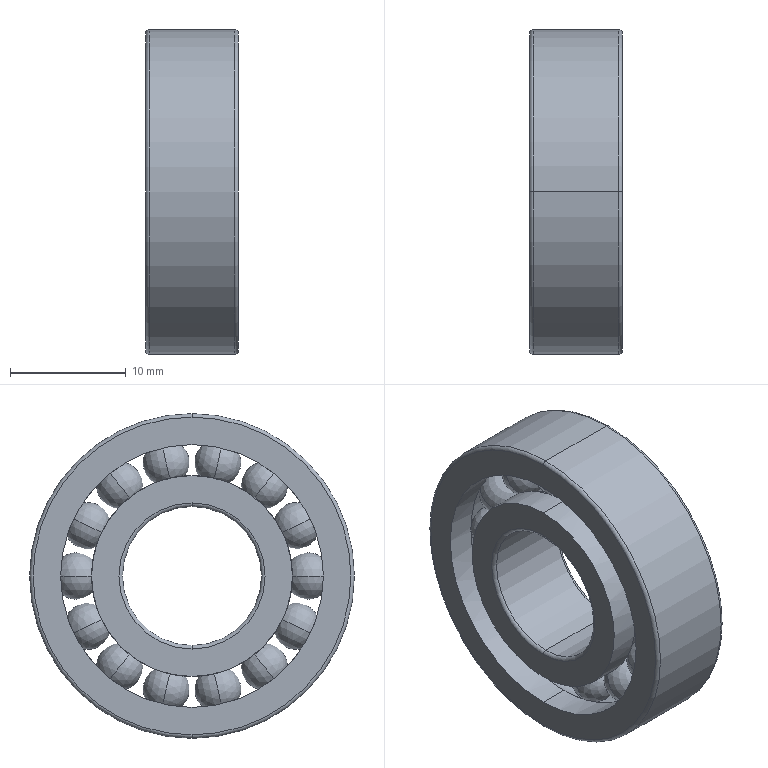Component | SolidWorks | GuideMechanism-1_SwingArm-1_Rolling bearings 6001 GB 276-94-1 | 1 solid | 97 faces | box 8 x 28 x 28 mm | volume 2976 mm3 | torus 53 | sphere 28 | cylinder 12 | plane 4 | commonest cylinder face diameters 22.667 x4 17.333 x4 28 x2 12 x2
build123d program:
from build123d import *

# Parameters (mm, degrees)
CIRCULAR_PATTERN1_COUNT = 14
FILLET1_R               = 0.3


with BuildPart() as part:
    # Sketch1 → Revolve1 (revolve)
    with BuildSketch(Plane.XY):
        with BuildLine():
            Line((-2, 10), (2, 10))
            ThreePointArc((2, 10), (0, 12), (-2, 10))
        make_face()
    revolve1 = revolve(axis=Axis((-4.597, 10, 0), (1, 0, 0)))

    # Sketch2 → Revolve2 (revolve)
    with BuildSketch(Plane.XY, mode=Mode.PRIVATE) as revolve2_sk:
        with BuildLine():
            Line((-4, 8.667), (-4, 6))
            Line((-4, 6), (4, 6))
            Line((4, 6), (4, 8.667))
            Line((4, 8.667), (1.477, 8.667))
            ThreePointArc((1.477, 8.667), (0, 8.01), (-1.477, 8.667))
            Line((-1.477, 8.667), (-4, 8.667))
        make_face()
    revolve(revolve2_sk.sketch.rotate(Axis((-6.971, 0, 0), (1, 0, 0)), 90), axis=Axis((-6.971, 0, 0), (1, 0, 0)))

    # Sketch3 → Revolve3 (revolve)
    with BuildSketch(Plane.XY, mode=Mode.PRIVATE) as revolve3_sk:
        with BuildLine():
            Line((-4, 14), (4, 14))
            Line((4, 14), (4, 11.333))
            Line((4, 11.333), (1.477, 11.333))
            ThreePointArc((1.477, 11.333), (0, 11.99), (-1.477, 11.333))
            Line((-1.477, 11.333), (-4, 11.333))
            Line((-4, 11.333), (-4, 14))
        make_face()
    revolve(revolve3_sk.sketch.rotate(Axis((-8.711, 0, 0), (1, 0, 0)), 90), axis=Axis((-8.711, 0, 0), (1, 0, 0)))

    # Circular-Pattern1: Revolve1 ×14 about axis
    circular_pattern1_axis = Axis((0, 0, 0), (1, 0, 0))
    for i in range(1, CIRCULAR_PATTERN1_COUNT):
        add(revolve1.rotate(circular_pattern1_axis, i * 360 / CIRCULAR_PATTERN1_COUNT))

    # Fillet1
    fillet1_edges = [part.edges().sort_by_distance(p)[0] for p in [
        (-4, 0, -14),
        (4, 0, -14),
        (-4, 0, -6),
        (4, 0, -6),
    ]]
    fillet(fillet1_edges, radius=FILLET1_R)


solid = part.part

# Placed as in the assembly
solid = solid.moved(Location((-591.272, -568.766, 1326.45), (0, 0, 0)))